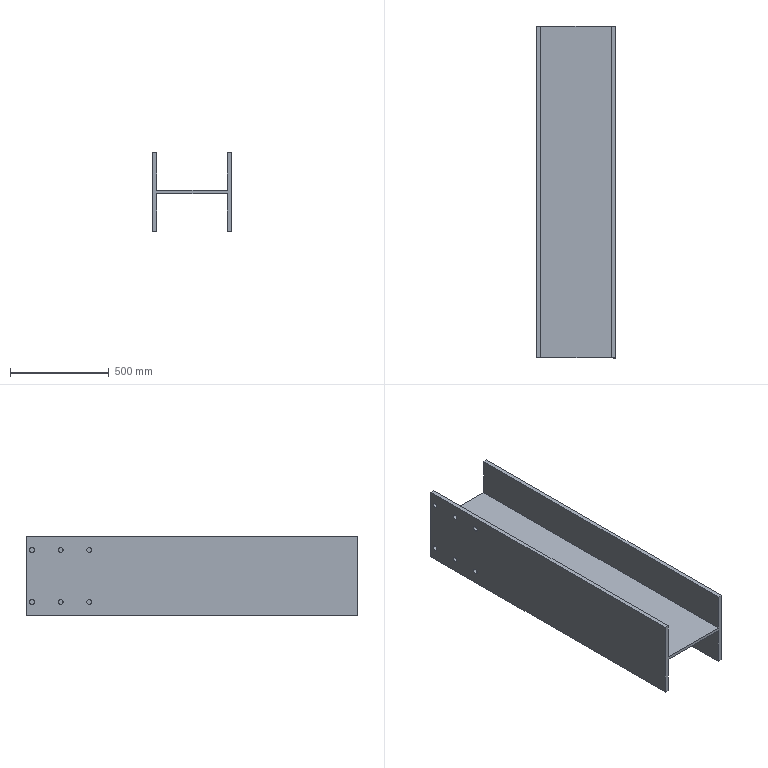Component | SolidWorks | I-Beam-5 | 1 solid | 26 faces | box 400 x 1680 x 400 mm | volume 37785190 mm3 | plane 14 | cylinder 12 | commonest cylinder face diameters 25 x12 | material Plain Carbon Steel
build123d program:
from build123d import *

# Parameters (mm, degrees)
BOSS_EXTRUDE1_DEPTH = 1680
CUT_EXTRUDE1_REACH  = 1774.682
SKETCH2_R           = 12.5


with BuildPart() as part:
    # Sketch1 → Boss-Extrude1 (new body)
    with BuildSketch(Plane(origin=(0, 0, 0), x_dir=(1, 0, 0), z_dir=(0, 1, 0))):
        Polygon((0, 0), (0, 400), (21, 400), (21, 208), (379, 208), (379, 400), (400, 400), (400, 0), (379, 0), (379, 192), (21, 192), (21, 0), align=None)
    extrude(amount=BOSS_EXTRUDE1_DEPTH)

    # Sketch2 → Cut-Extrude1 (cut, up to next)
    with BuildSketch(Plane(origin=(400, 0, 0), x_dir=(0, 0, -1), z_dir=(1, 0, 0)), mode=Mode.PRIVATE) as cut_extrude1_sk1:
        with Locations((68.182, 1650)):
            Circle(SKETCH2_R)
    cut_extrude1_tool1 = extrude(cut_extrude1_sk1.sketch, amount=-CUT_EXTRUDE1_REACH, mode=Mode.PRIVATE) & part.part
    # Sketch2 → Cut-Extrude1 (cut, up to next)
    with BuildSketch(Plane(origin=(400, 0, 0), x_dir=(0, 0, -1), z_dir=(1, 0, 0)), mode=Mode.PRIVATE) as cut_extrude1_sk2:
        with Locations((68.182, 1505)):
            Circle(SKETCH2_R)
    cut_extrude1_tool2 = extrude(cut_extrude1_sk2.sketch, amount=-CUT_EXTRUDE1_REACH, mode=Mode.PRIVATE) & part.part
    # Sketch2 → Cut-Extrude1 (cut, up to next)
    with BuildSketch(Plane(origin=(400, 0, 0), x_dir=(0, 0, -1), z_dir=(1, 0, 0)), mode=Mode.PRIVATE) as cut_extrude1_sk3:
        with Locations((331.818, 1360)):
            Circle(SKETCH2_R)
    cut_extrude1_tool3 = extrude(cut_extrude1_sk3.sketch, amount=-CUT_EXTRUDE1_REACH, mode=Mode.PRIVATE) & part.part
    # Sketch2 → Cut-Extrude1 (cut, up to next)
    with BuildSketch(Plane(origin=(400, 0, 0), x_dir=(0, 0, -1), z_dir=(1, 0, 0)), mode=Mode.PRIVATE) as cut_extrude1_sk4:
        with Locations((331.818, 1505)):
            Circle(SKETCH2_R)
    cut_extrude1_tool4 = extrude(cut_extrude1_sk4.sketch, amount=-CUT_EXTRUDE1_REACH, mode=Mode.PRIVATE) & part.part
    # Sketch2 → Cut-Extrude1 (cut, up to next)
    with BuildSketch(Plane(origin=(400, 0, 0), x_dir=(0, 0, -1), z_dir=(1, 0, 0)), mode=Mode.PRIVATE) as cut_extrude1_sk5:
        with Locations((331.818, 1650)):
            Circle(SKETCH2_R)
    cut_extrude1_tool5 = extrude(cut_extrude1_sk5.sketch, amount=-CUT_EXTRUDE1_REACH, mode=Mode.PRIVATE) & part.part
    # Sketch2 → Cut-Extrude1 (cut, up to next)
    with BuildSketch(Plane(origin=(400, 0, 0), x_dir=(0, 0, -1), z_dir=(1, 0, 0)), mode=Mode.PRIVATE) as cut_extrude1_sk6:
        with Locations((68.182, 1360)):
            Circle(SKETCH2_R)
    cut_extrude1_tool6 = extrude(cut_extrude1_sk6.sketch, amount=-CUT_EXTRUDE1_REACH, mode=Mode.PRIVATE) & part.part
    add(cut_extrude1_tool1.solids().sort_by_distance((400, 1650, -68.182))[0], mode=Mode.SUBTRACT)
    add(cut_extrude1_tool2.solids().sort_by_distance((400, 1505, -68.182))[0], mode=Mode.SUBTRACT)
    add(cut_extrude1_tool3.solids().sort_by_distance((400, 1360, -331.818))[0], mode=Mode.SUBTRACT)
    add(cut_extrude1_tool4.solids().sort_by_distance((400, 1505, -331.818))[0], mode=Mode.SUBTRACT)
    add(cut_extrude1_tool5.solids().sort_by_distance((400, 1650, -331.818))[0], mode=Mode.SUBTRACT)
    add(cut_extrude1_tool6.solids().sort_by_distance((400, 1360, -68.182))[0], mode=Mode.SUBTRACT)


solid = part.part

# Placed as in the assembly
solid = solid.moved(Location((17054.937, 1194.803, 1655.287), (-180, 0, 180)))
STEP:
#1=COLOUR_RGB('',0.7922,0.8196,0.9333);
#2=FILL_AREA_STYLE_COLOUR('',#1);
#3=FILL_AREA_STYLE('',(#2));
#4=SURFACE_STYLE_FILL_AREA(#3);
#5=SURFACE_SIDE_STYLE('',(#4));
#6=SURFACE_STYLE_USAGE(.BOTH.,#5);
#7=PRESENTATION_STYLE_ASSIGNMENT((#6));
#8=CARTESIAN_POINT('',(656.533,100.583,68.345));
#9=VERTEX_POINT('',#8);
#10=CARTESIAN_POINT('',(656.533,100.583,67.361));
#11=VERTEX_POINT('',#10);
#12=CARTESIAN_POINT('',(656.533,100.583,67.853));
#13=DIRECTION('',(1.,-0.,-0.));
#14=DIRECTION('',(0.,0.,1.));
#15=AXIS2_PLACEMENT_3D('',#12,#13,#14);
#16=CIRCLE('',#15,0.4921);
#17=EDGE_CURVE('',#9,#11,#16,.T.);
#18=ORIENTED_EDGE('',*,*,#17,.T.);
#19=CARTESIAN_POINT('',(655.706,100.583,67.361));
#20=VERTEX_POINT('',#19);
#21=CARTESIAN_POINT('',(671.454,100.583,67.361));
#22=DIRECTION('',(-1.,0.,0.));
#23=VECTOR('',#22,39.37);
#24=LINE('',#21,#23);
#25=EDGE_CURVE('',#11,#20,#24,.T.);
#26=ORIENTED_EDGE('',*,*,#25,.T.);
#27=CARTESIAN_POINT('',(655.706,100.583,68.345));
#28=VERTEX_POINT('',#27);
#29=CARTESIAN_POINT('',(655.706,100.583,67.853));
#30=DIRECTION('',(-1.,0.,0.));
#31=DIRECTION('',(0.,0.,1.));
#32=AXIS2_PLACEMENT_3D('',#29,#30,#31);
#33=CIRCLE('',#32,0.4921);
#34=EDGE_CURVE('',#20,#28,#33,.T.);
#35=ORIENTED_EDGE('',*,*,#34,.T.);
#36=CARTESIAN_POINT('',(671.454,100.583,68.345));
#37=DIRECTION('',(-1.,0.,0.));
#38=VECTOR('',#37,39.37);
#39=LINE('',#36,#38);
#40=EDGE_CURVE('',#9,#28,#39,.T.);
#41=ORIENTED_EDGE('',*,*,#40,.F.);
#42=EDGE_LOOP('',(#18,#26,#35,#41));
#43=FACE_OUTER_BOUND('',#42,.T.);
#44=CARTESIAN_POINT('',(671.454,100.583,67.853));
#45=DIRECTION('',(-1.,0.,0.));
#46=DIRECTION('',(0.,0.,1.));
#47=AXIS2_PLACEMENT_3D('',#44,#45,#46);
#48=CYLINDRICAL_SURFACE('',#47,0.4921);
#49=ADVANCED_FACE('',(#43),#48,.F.);
#50=CARTESIAN_POINT('',(656.533,106.291,68.345));
#51=VERTEX_POINT('',#50);
#52=CARTESIAN_POINT('',(656.533,106.291,67.361));
#53=VERTEX_POINT('',#52);
#54=CARTESIAN_POINT('',(656.533,106.291,67.853));
#55=DIRECTION('',(1.,-0.,-0.));
#56=DIRECTION('',(0.,0.,1.));
#57=AXIS2_PLACEMENT_3D('',#54,#55,#56);
#58=CIRCLE('',#57,0.4921);
#59=EDGE_CURVE('',#51,#53,#58,.T.);
#60=ORIENTED_EDGE('',*,*,#59,.T.);
#61=CARTESIAN_POINT('',(655.706,106.291,67.361));
#62=VERTEX_POINT('',#61);
#63=CARTESIAN_POINT('',(671.454,106.291,67.361));
#64=DIRECTION('',(-1.,0.,0.));
#65=VECTOR('',#64,39.37);
#66=LINE('',#63,#65);
#67=EDGE_CURVE('',#53,#62,#66,.T.);
#68=ORIENTED_EDGE('',*,*,#67,.T.);
#69=CARTESIAN_POINT('',(655.706,106.291,68.345));
#70=VERTEX_POINT('',#69);
#71=CARTESIAN_POINT('',(655.706,106.291,67.853));
#72=DIRECTION('',(-1.,0.,0.));
#73=DIRECTION('',(0.,0.,1.));
#74=AXIS2_PLACEMENT_3D('',#71,#72,#73);
#75=CIRCLE('',#74,0.4921);
#76=EDGE_CURVE('',#62,#70,#75,.T.);
#77=ORIENTED_EDGE('',*,*,#76,.T.);
#78=CARTESIAN_POINT('',(671.454,106.291,68.345));
#79=DIRECTION('',(-1.,0.,0.));
#80=VECTOR('',#79,39.37);
#81=LINE('',#78,#80);
#82=EDGE_CURVE('',#51,#70,#81,.T.);
#83=ORIENTED_EDGE('',*,*,#82,.F.);
#84=EDGE_LOOP('',(#60,#68,#77,#83));
#85=FACE_OUTER_BOUND('',#84,.T.);
#86=CARTESIAN_POINT('',(671.454,106.291,67.853));
#87=DIRECTION('',(-1.,0.,0.));
#88=DIRECTION('',(0.,0.,1.));
#89=AXIS2_PLACEMENT_3D('',#86,#87,#88);
#90=CYLINDRICAL_SURFACE('',#89,0.4921);
#91=ADVANCED_FACE('',(#85),#90,.F.);
#92=CARTESIAN_POINT('',(656.533,112.,68.345));
#93=VERTEX_POINT('',#92);
#94=CARTESIAN_POINT('',(656.533,112.,67.361));
#95=VERTEX_POINT('',#94);
#96=CARTESIAN_POINT('',(656.533,112.,67.853));
#97=DIRECTION('',(1.,-0.,-0.));
#98=DIRECTION('',(0.,0.,1.));
#99=AXIS2_PLACEMENT_3D('',#96,#97,#98);
#100=CIRCLE('',#99,0.4921);
#101=EDGE_CURVE('',#93,#95,#100,.T.);
#102=ORIENTED_EDGE('',*,*,#101,.T.);
#103=CARTESIAN_POINT('',(655.706,112.,67.361));
#104=VERTEX_POINT('',#103);
#105=CARTESIAN_POINT('',(671.454,112.,67.361));
#106=DIRECTION('',(-1.,0.,0.));
#107=VECTOR('',#106,39.37);
#108=LINE('',#105,#107);
#109=EDGE_CURVE('',#95,#104,#108,.T.);
#110=ORIENTED_EDGE('',*,*,#109,.T.);
#111=CARTESIAN_POINT('',(655.706,112.,68.345));
#112=VERTEX_POINT('',#111);
#113=CARTESIAN_POINT('',(655.706,112.,67.853));
#114=DIRECTION('',(-1.,0.,0.));
#115=DIRECTION('',(0.,0.,1.));
#116=AXIS2_PLACEMENT_3D('',#113,#114,#115);
#117=CIRCLE('',#116,0.4921);
#118=EDGE_CURVE('',#104,#112,#117,.T.);
#119=ORIENTED_EDGE('',*,*,#118,.T.);
#120=CARTESIAN_POINT('',(671.454,112.,68.345));
#121=DIRECTION('',(-1.,0.,0.));
#122=VECTOR('',#121,39.37);
#123=LINE('',#120,#122);
#124=EDGE_CURVE('',#93,#112,#123,.T.);
#125=ORIENTED_EDGE('',*,*,#124,.F.);
#126=EDGE_LOOP('',(#102,#110,#119,#125));
#127=FACE_OUTER_BOUND('',#126,.T.);
#128=CARTESIAN_POINT('',(671.454,112.,67.853));
#129=DIRECTION('',(-1.,0.,0.));
#130=DIRECTION('',(0.,0.,1.));
#131=AXIS2_PLACEMENT_3D('',#128,#129,#130);
#132=CYLINDRICAL_SURFACE('',#131,0.4921);
#133=ADVANCED_FACE('',(#127),#132,.F.);
#134=CARTESIAN_POINT('',(656.533,112.,78.725));
#135=VERTEX_POINT('',#134);
#136=CARTESIAN_POINT('',(656.533,112.,77.74));
#137=VERTEX_POINT('',#136);
#138=CARTESIAN_POINT('',(656.533,112.,78.232));
#139=DIRECTION('',(1.,-0.,-0.));
#140=DIRECTION('',(0.,0.,1.));
#141=AXIS2_PLACEMENT_3D('',#138,#139,#140);
#142=CIRCLE('',#141,0.4921);
#143=EDGE_CURVE('',#135,#137,#142,.T.);
#144=ORIENTED_EDGE('',*,*,#143,.T.);
#145=CARTESIAN_POINT('',(655.706,112.,77.74));
#146=VERTEX_POINT('',#145);
#147=CARTESIAN_POINT('',(671.454,112.,77.74));
#148=DIRECTION('',(-1.,0.,0.));
#149=VECTOR('',#148,39.37);
#150=LINE('',#147,#149);
#151=EDGE_CURVE('',#137,#146,#150,.T.);
#152=ORIENTED_EDGE('',*,*,#151,.T.);
#153=CARTESIAN_POINT('',(655.706,112.,78.725));
#154=VERTEX_POINT('',#153);
#155=CARTESIAN_POINT('',(655.706,112.,78.232));
#156=DIRECTION('',(-1.,0.,0.));
#157=DIRECTION('',(0.,0.,1.));
#158=AXIS2_PLACEMENT_3D('',#155,#156,#157);
#159=CIRCLE('',#158,0.4921);
#160=EDGE_CURVE('',#146,#154,#159,.T.);
#161=ORIENTED_EDGE('',*,*,#160,.T.);
#162=CARTESIAN_POINT('',(671.454,112.,78.725));
#163=DIRECTION('',(-1.,0.,0.));
#164=VECTOR('',#163,39.37);
#165=LINE('',#162,#164);
#166=EDGE_CURVE('',#135,#154,#165,.T.);
#167=ORIENTED_EDGE('',*,*,#166,.F.);
#168=EDGE_LOOP('',(#144,#152,#161,#167));
#169=FACE_OUTER_BOUND('',#168,.T.);
#170=CARTESIAN_POINT('',(671.454,112.,78.232));
#171=DIRECTION('',(-1.,0.,0.));
#172=DIRECTION('',(0.,0.,1.));
#173=AXIS2_PLACEMENT_3D('',#170,#171,#172);
#174=CYLINDRICAL_SURFACE('',#173,0.4921);
#175=ADVANCED_FACE('',(#169),#174,.F.);
#176=CARTESIAN_POINT('',(656.533,106.291,78.725));
#177=VERTEX_POINT('',#176);
#178=CARTESIAN_POINT('',(656.533,106.291,77.74));
#179=VERTEX_POINT('',#178);
#180=CARTESIAN_POINT('',(656.533,106.291,78.232));
#181=DIRECTION('',(1.,-0.,-0.));
#182=DIRECTION('',(0.,0.,1.));
#183=AXIS2_PLACEMENT_3D('',#180,#181,#182);
#184=CIRCLE('',#183,0.4921);
#185=EDGE_CURVE('',#177,#179,#184,.T.);
#186=ORIENTED_EDGE('',*,*,#185,.T.);
#187=CARTESIAN_POINT('',(655.706,106.291,77.74));
#188=VERTEX_POINT('',#187);
#189=CARTESIAN_POINT('',(671.454,106.291,77.74));
#190=DIRECTION('',(-1.,0.,0.));
#191=VECTOR('',#190,39.37);
#192=LINE('',#189,#191);
#193=EDGE_CURVE('',#179,#188,#192,.T.);
#194=ORIENTED_EDGE('',*,*,#193,.T.);
#195=CARTESIAN_POINT('',(655.706,106.291,78.725));
#196=VERTEX_POINT('',#195);
#197=CARTESIAN_POINT('',(655.706,106.291,78.232));
#198=DIRECTION('',(-1.,0.,0.));
#199=DIRECTION('',(0.,0.,1.));
#200=AXIS2_PLACEMENT_3D('',#197,#198,#199);
#201=CIRCLE('',#200,0.4921);
#202=EDGE_CURVE('',#188,#196,#201,.T.);
#203=ORIENTED_EDGE('',*,*,#202,.T.);
#204=CARTESIAN_POINT('',(671.454,106.291,78.725));
#205=DIRECTION('',(-1.,0.,0.));
#206=VECTOR('',#205,39.37);
#207=LINE('',#204,#206);
#208=EDGE_CURVE('',#177,#196,#207,.T.);
#209=ORIENTED_EDGE('',*,*,#208,.F.);
#210=EDGE_LOOP('',(#186,#194,#203,#209));
#211=FACE_OUTER_BOUND('',#210,.T.);
#212=CARTESIAN_POINT('',(671.454,106.291,78.232));
#213=DIRECTION('',(-1.,0.,0.));
#214=DIRECTION('',(0.,0.,1.));
#215=AXIS2_PLACEMENT_3D('',#212,#213,#214);
#216=CYLINDRICAL_SURFACE('',#215,0.4921);
#217=ADVANCED_FACE('',(#211),#216,.F.);
#218=CARTESIAN_POINT('',(656.533,100.583,78.725));
#219=VERTEX_POINT('',#218);
#220=CARTESIAN_POINT('',(656.533,100.583,77.74));
#221=VERTEX_POINT('',#220);
#222=CARTESIAN_POINT('',(656.533,100.583,78.232));
#223=DIRECTION('',(1.,-0.,-0.));
#224=DIRECTION('',(0.,0.,1.));
#225=AXIS2_PLACEMENT_3D('',#222,#223,#224);
#226=CIRCLE('',#225,0.4921);
#227=EDGE_CURVE('',#219,#221,#226,.T.);
#228=ORIENTED_EDGE('',*,*,#227,.T.);
#229=CARTESIAN_POINT('',(655.706,100.583,77.74));
#230=VERTEX_POINT('',#229);
#231=CARTESIAN_POINT('',(671.454,100.583,77.74));
#232=DIRECTION('',(-1.,0.,0.));
#233=VECTOR('',#232,39.37);
#234=LINE('',#231,#233);
#235=EDGE_CURVE('',#221,#230,#234,.T.);
#236=ORIENTED_EDGE('',*,*,#235,.T.);
#237=CARTESIAN_POINT('',(655.706,100.583,78.725));
#238=VERTEX_POINT('',#237);
#239=CARTESIAN_POINT('',(655.706,100.583,78.232));
#240=DIRECTION('',(-1.,0.,0.));
#241=DIRECTION('',(0.,0.,1.));
#242=AXIS2_PLACEMENT_3D('',#239,#240,#241);
#243=CIRCLE('',#242,0.4921);
#244=EDGE_CURVE('',#230,#238,#243,.T.);
#245=ORIENTED_EDGE('',*,*,#244,.T.);
#246=CARTESIAN_POINT('',(671.454,100.583,78.725));
#247=DIRECTION('',(-1.,0.,0.));
#248=VECTOR('',#247,39.37);
#249=LINE('',#246,#248);
#250=EDGE_CURVE('',#219,#238,#249,.T.);
#251=ORIENTED_EDGE('',*,*,#250,.F.);
#252=EDGE_LOOP('',(#228,#236,#245,#251));
#253=FACE_OUTER_BOUND('',#252,.T.);
#254=CARTESIAN_POINT('',(671.454,100.583,78.232));
#255=DIRECTION('',(-1.,0.,0.));
#256=DIRECTION('',(0.,0.,1.));
#257=AXIS2_PLACEMENT_3D('',#254,#255,#256);
#258=CYLINDRICAL_SURFACE('',#257,0.4921);
#259=ADVANCED_FACE('',(#253),#258,.F.);
#260=CARTESIAN_POINT('',(671.454,47.039,65.169));
#261=VERTEX_POINT('',#260);
#262=CARTESIAN_POINT('',(670.627,47.039,65.169));
#263=VERTEX_POINT('',#262);
#264=CARTESIAN_POINT('',(670.627,47.039,65.169));
#265=DIRECTION('',(-1.,0.,0.));
#266=VECTOR('',#265,39.37);
#267=LINE('',#264,#266);
#268=EDGE_CURVE('',#261,#263,#267,.T.);
#269=ORIENTED_EDGE('',*,*,#268,.T.);
#270=CARTESIAN_POINT('',(670.627,113.181,65.169));
#271=VERTEX_POINT('',#270);
#272=CARTESIAN_POINT('',(670.627,113.181,65.169));
#273=DIRECTION('',(-0.,-1.,0.));
#274=VECTOR('',#273,39.37);
#275=LINE('',#272,#274);
#276=EDGE_CURVE('',#271,#263,#275,.T.);
#277=ORIENTED_EDGE('',*,*,#276,.F.);
#278=CARTESIAN_POINT('',(671.454,113.181,65.169));
#279=VERTEX_POINT('',#278);
#280=CARTESIAN_POINT('',(670.627,113.181,65.169));
#281=DIRECTION('',(-1.,0.,0.));
#282=VECTOR('',#281,39.37);
#283=LINE('',#280,#282);
#284=EDGE_CURVE('',#279,#271,#283,.T.);
#285=ORIENTED_EDGE('',*,*,#284,.F.);
#286=CARTESIAN_POINT('',(671.454,113.181,65.169));
#287=DIRECTION('',(-0.,-1.,0.));
#288=VECTOR('',#287,39.37);
#289=LINE('',#286,#288);
#290=EDGE_CURVE('',#279,#261,#289,.T.);
#291=ORIENTED_EDGE('',*,*,#290,.T.);
#292=EDGE_LOOP('',(#269,#277,#285,#291));
#293=FACE_OUTER_BOUND('',#292,.T.);
#294=CARTESIAN_POINT('',(670.627,113.181,65.169));
#295=DIRECTION('',(0.,-0.,1.));
#296=DIRECTION('',(1.,-0.,-0.));
#297=AXIS2_PLACEMENT_3D('',#294,#295,#296);
#298=PLANE('',#297);
#299=ADVANCED_FACE('',(#293),#298,.F.);
#300=CARTESIAN_POINT('',(670.627,47.039,72.728));
#301=VERTEX_POINT('',#300);
#302=CARTESIAN_POINT('',(670.627,47.039,72.728));
#303=DIRECTION('',(0.,-0.,1.));
#304=VECTOR('',#303,39.37);
#305=LINE('',#302,#304);
#306=EDGE_CURVE('',#263,#301,#305,.T.);
#307=ORIENTED_EDGE('',*,*,#306,.T.);
#308=CARTESIAN_POINT('',(670.627,113.181,72.728));
#309=VERTEX_POINT('',#308);
#310=CARTESIAN_POINT('',(670.627,113.181,72.728));
#311=DIRECTION('',(-0.,-1.,0.));
#312=VECTOR('',#311,39.37);
#313=LINE('',#310,#312);
#314=EDGE_CURVE('',#309,#301,#313,.T.);
#315=ORIENTED_EDGE('',*,*,#314,.F.);
#316=CARTESIAN_POINT('',(670.627,113.181,72.728));
#317=DIRECTION('',(0.,-0.,1.));
#318=VECTOR('',#317,39.37);
#319=LINE('',#316,#318);
#320=EDGE_CURVE('',#271,#309,#319,.T.);
#321=ORIENTED_EDGE('',*,*,#320,.F.);
#322=ORIENTED_EDGE('',*,*,#276,.T.);
#323=EDGE_LOOP('',(#307,#315,#321,#322));
#324=FACE_OUTER_BOUND('',#323,.T.);
#325=CARTESIAN_POINT('',(670.627,113.181,72.728));
#326=DIRECTION('',(1.,-0.,-0.));
#327=DIRECTION('',(-0.,0.,-1.));
#328=AXIS2_PLACEMENT_3D('',#325,#326,#327);
#329=PLANE('',#328);
#330=ADVANCED_FACE('',(#324),#329,.F.);
#331=CARTESIAN_POINT('',(656.533,47.039,72.728));
#332=VERTEX_POINT('',#331);
#333=CARTESIAN_POINT('',(656.533,47.039,72.728));
#334=DIRECTION('',(-1.,0.,0.));
#335=VECTOR('',#334,39.37);
#336=LINE('',#333,#335);
#337=EDGE_CURVE('',#301,#332,#336,.T.);
#338=ORIENTED_EDGE('',*,*,#337,.T.);
#339=CARTESIAN_POINT('',(656.533,113.181,72.728));
#340=VERTEX_POINT('',#339);
#341=CARTESIAN_POINT('',(656.533,113.181,72.728));
#342=DIRECTION('',(-0.,-1.,0.));
#343=VECTOR('',#342,39.37);
#344=LINE('',#341,#343);
#345=EDGE_CURVE('',#340,#332,#344,.T.);
#346=ORIENTED_EDGE('',*,*,#345,.F.);
#347=CARTESIAN_POINT('',(656.533,113.181,72.728));
#348=DIRECTION('',(-1.,0.,0.));
#349=VECTOR('',#348,39.37);
#350=LINE('',#347,#349);
#351=EDGE_CURVE('',#309,#340,#350,.T.);
#352=ORIENTED_EDGE('',*,*,#351,.F.);
#353=ORIENTED_EDGE('',*,*,#314,.T.);
#354=EDGE_LOOP('',(#338,#346,#352,#353));
#355=FACE_OUTER_BOUND('',#354,.T.);
#356=CARTESIAN_POINT('',(656.533,113.181,72.728));
#357=DIRECTION('',(0.,-0.,1.));
#358=DIRECTION('',(1.,-0.,-0.));
#359=AXIS2_PLACEMENT_3D('',#356,#357,#358);
#360=PLANE('',#359);
#361=ADVANCED_FACE('',(#355),#360,.F.);
#362=ORIENTED_EDGE('',*,*,#17,.F.);
#363=CARTESIAN_POINT('',(656.533,100.583,67.853));
#364=DIRECTION('',(1.,-0.,-0.));
#365=DIRECTION('',(0.,0.,1.));
#366=AXIS2_PLACEMENT_3D('',#363,#364,#365);
#367=CIRCLE('',#366,0.4921);
#368=EDGE_CURVE('',#11,#9,#367,.T.);
#369=ORIENTED_EDGE('',*,*,#368,.F.);
#370=EDGE_LOOP('',(#362,#369));
#371=FACE_BOUND('',#370,.T.);
#372=ORIENTED_EDGE('',*,*,#59,.F.);
#373=CARTESIAN_POINT('',(656.533,106.291,67.853));
#374=DIRECTION('',(1.,-0.,-0.));
#375=DIRECTION('',(0.,0.,1.));
#376=AXIS2_PLACEMENT_3D('',#373,#374,#375);
#377=CIRCLE('',#376,0.4921);
#378=EDGE_CURVE('',#53,#51,#377,.T.);
#379=ORIENTED_EDGE('',*,*,#378,.F.);
#380=EDGE_LOOP('',(#372,#379));
#381=FACE_BOUND('',#380,.T.);
#382=ORIENTED_EDGE('',*,*,#101,.F.);
#383=CARTESIAN_POINT('',(656.533,112.,67.853));
#384=DIRECTION('',(1.,-0.,-0.));
#385=DIRECTION('',(0.,0.,1.));
#386=AXIS2_PLACEMENT_3D('',#383,#384,#385);
#387=CIRCLE('',#386,0.4921);
#388=EDGE_CURVE('',#95,#93,#387,.T.);
#389=ORIENTED_EDGE('',*,*,#388,.F.);
#390=EDGE_LOOP('',(#382,#389));
#391=FACE_BOUND('',#390,.T.);
#392=CARTESIAN_POINT('',(656.533,47.039,65.169));
#393=VERTEX_POINT('',#392);
#394=CARTESIAN_POINT('',(656.533,47.039,65.169));
#395=DIRECTION('',(-0.,0.,-1.));
#396=VECTOR('',#395,39.37);
#397=LINE('',#394,#396);
#398=EDGE_CURVE('',#332,#393,#397,.T.);
#399=ORIENTED_EDGE('',*,*,#398,.T.);
#400=CARTESIAN_POINT('',(656.533,113.181,65.169));
#401=VERTEX_POINT('',#400);
#402=CARTESIAN_POINT('',(656.533,113.181,65.169));
#403=DIRECTION('',(-0.,-1.,0.));
#404=VECTOR('',#403,39.37);
#405=LINE('',#402,#404);
#406=EDGE_CURVE('',#401,#393,#405,.T.);
#407=ORIENTED_EDGE('',*,*,#406,.F.);
#408=CARTESIAN_POINT('',(656.533,113.181,65.169));
#409=DIRECTION('',(-0.,0.,-1.));
#410=VECTOR('',#409,39.37);
#411=LINE('',#408,#410);
#412=EDGE_CURVE('',#340,#401,#411,.T.);
#413=ORIENTED_EDGE('',*,*,#412,.F.);
#414=ORIENTED_EDGE('',*,*,#345,.T.);
#415=EDGE_LOOP('',(#399,#407,#413,#414));
#416=FACE_OUTER_BOUND('',#415,.T.);
#417=CARTESIAN_POINT('',(656.533,113.181,65.169));
#418=DIRECTION('',(-1.,0.,0.));
#419=DIRECTION('',(0.,-0.,1.));
#420=AXIS2_PLACEMENT_3D('',#417,#418,#419);
#421=PLANE('',#420);
#422=ADVANCED_FACE('',(#371,#381,#391,#416),#421,.F.);
#423=CARTESIAN_POINT('',(655.706,47.039,65.169));
#424=VERTEX_POINT('',#423);
#425=CARTESIAN_POINT('',(655.706,47.039,65.169));
#426=DIRECTION('',(-1.,0.,0.));
#427=VECTOR('',#426,39.37);
#428=LINE('',#425,#427);
#429=EDGE_CURVE('',#393,#424,#428,.T.);
#430=ORIENTED_EDGE('',*,*,#429,.T.);
#431=CARTESIAN_POINT('',(655.706,113.181,65.169));
#432=VERTEX_POINT('',#431);
#433=CARTESIAN_POINT('',(655.706,113.181,65.169));
#434=DIRECTION('',(-0.,-1.,0.));
#435=VECTOR('',#434,39.37);
#436=LINE('',#433,#435);
#437=EDGE_CURVE('',#432,#424,#436,.T.);
#438=ORIENTED_EDGE('',*,*,#437,.F.);
#439=CARTESIAN_POINT('',(655.706,113.181,65.169));
#440=DIRECTION('',(-1.,0.,0.));
#441=VECTOR('',#440,39.37);
#442=LINE('',#439,#441);
#443=EDGE_CURVE('',#401,#432,#442,.T.);
#444=ORIENTED_EDGE('',*,*,#443,.F.);
#445=ORIENTED_EDGE('',*,*,#406,.T.);
#446=EDGE_LOOP('',(#430,#438,#444,#445));
#447=FACE_OUTER_BOUND('',#446,.T.);
#448=CARTESIAN_POINT('',(655.706,113.181,65.169));
#449=DIRECTION('',(0.,-0.,1.));
#450=DIRECTION('',(1.,-0.,-0.));
#451=AXIS2_PLACEMENT_3D('',#448,#449,#450);
#452=PLANE('',#451);
#453=ADVANCED_FACE('',(#447),#452,.F.);
#454=CARTESIAN_POINT('',(655.706,112.,78.232));
#455=DIRECTION('',(-1.,0.,0.));
#456=DIRECTION('',(0.,0.,1.));
#457=AXIS2_PLACEMENT_3D('',#454,#455,#456);
#458=CIRCLE('',#457,0.4921);
#459=EDGE_CURVE('',#154,#146,#458,.T.);
#460=ORIENTED_EDGE('',*,*,#459,.F.);
#461=ORIENTED_EDGE('',*,*,#160,.F.);
#462=EDGE_LOOP('',(#460,#461));
#463=FACE_BOUND('',#462,.T.);
#464=CARTESIAN_POINT('',(655.706,106.291,78.232));
#465=DIRECTION('',(-1.,0.,0.));
#466=DIRECTION('',(0.,0.,1.));
#467=AXIS2_PLACEMENT_3D('',#464,#465,#466);
#468=CIRCLE('',#467,0.4921);
#469=EDGE_CURVE('',#196,#188,#468,.T.);
#470=ORIENTED_EDGE('',*,*,#469,.F.);
#471=ORIENTED_EDGE('',*,*,#202,.F.);
#472=EDGE_LOOP('',(#470,#471));
#473=FACE_BOUND('',#472,.T.);
#474=CARTESIAN_POINT('',(655.706,100.583,78.232));
#475=DIRECTION('',(-1.,0.,0.));
#476=DIRECTION('',(0.,0.,1.));
#477=AXIS2_PLACEMENT_3D('',#474,#475,#476);
#478=CIRCLE('',#477,0.4921);
#479=EDGE_CURVE('',#238,#230,#478,.T.);
#480=ORIENTED_EDGE('',*,*,#479,.F.);
#481=ORIENTED_EDGE('',*,*,#244,.F.);
#482=EDGE_LOOP('',(#480,#481));
#483=FACE_BOUND('',#482,.T.);
#484=CARTESIAN_POINT('',(655.706,100.583,67.853));
#485=DIRECTION('',(-1.,0.,0.));
#486=DIRECTION('',(0.,0.,1.));
#487=AXIS2_PLACEMENT_3D('',#484,#485,#486);
#488=CIRCLE('',#487,0.4921);
#489=EDGE_CURVE('',#28,#20,#488,.T.);
#490=ORIENTED_EDGE('',*,*,#489,.F.);
#491=ORIENTED_EDGE('',*,*,#34,.F.);
#492=EDGE_LOOP('',(#490,#491));
#493=FACE_BOUND('',#492,.T.);
#494=CARTESIAN_POINT('',(655.706,106.291,67.853));
#495=DIRECTION('',(-1.,0.,0.));
#496=DIRECTION('',(0.,0.,1.));
#497=AXIS2_PLACEMENT_3D('',#494,#495,#496);
#498=CIRCLE('',#497,0.4921);
#499=EDGE_CURVE('',#70,#62,#498,.T.);
#500=ORIENTED_EDGE('',*,*,#499,.F.);
#501=ORIENTED_EDGE('',*,*,#76,.F.);
#502=EDGE_LOOP('',(#500,#501));
#503=FACE_BOUND('',#502,.T.);
#504=CARTESIAN_POINT('',(655.706,112.,67.853));
#505=DIRECTION('',(-1.,0.,0.));
#506=DIRECTION('',(0.,0.,1.));
#507=AXIS2_PLACEMENT_3D('',#504,#505,#506);
#508=CIRCLE('',#507,0.4921);
#509=EDGE_CURVE('',#112,#104,#508,.T.);
#510=ORIENTED_EDGE('',*,*,#509,.F.);
#511=ORIENTED_EDGE('',*,*,#118,.F.);
#512=EDGE_LOOP('',(#510,#511));
#513=FACE_BOUND('',#512,.T.);
#514=CARTESIAN_POINT('',(655.706,47.039,80.917));
#515=VERTEX_POINT('',#514);
#516=CARTESIAN_POINT('',(655.706,47.039,80.917));
#517=DIRECTION('',(0.,-0.,1.));
#518=VECTOR('',#517,39.37);
#519=LINE('',#516,#518);
#520=EDGE_CURVE('',#424,#515,#519,.T.);
#521=ORIENTED_EDGE('',*,*,#520,.T.);
#522=CARTESIAN_POINT('',(655.706,113.181,80.917));
#523=VERTEX_POINT('',#522);
#524=CARTESIAN_POINT('',(655.706,113.181,80.917));
#525=DIRECTION('',(-0.,-1.,0.));
#526=VECTOR('',#525,39.37);
#527=LINE('',#524,#526);
#528=EDGE_CURVE('',#523,#515,#527,.T.);
#529=ORIENTED_EDGE('',*,*,#528,.F.);
#530=CARTESIAN_POINT('',(655.706,113.181,80.917));
#531=DIRECTION('',(0.,-0.,1.));
#532=VECTOR('',#531,39.37);
#533=LINE('',#530,#532);
#534=EDGE_CURVE('',#432,#523,#533,.T.);
#535=ORIENTED_EDGE('',*,*,#534,.F.);
#536=ORIENTED_EDGE('',*,*,#437,.T.);
#537=EDGE_LOOP('',(#521,#529,#535,#536));
#538=FACE_OUTER_BOUND('',#537,.T.);
#539=CARTESIAN_POINT('',(655.706,113.181,80.917));
#540=DIRECTION('',(1.,-0.,-0.));
#541=DIRECTION('',(-0.,0.,-1.));
#542=AXIS2_PLACEMENT_3D('',#539,#540,#541);
#543=PLANE('',#542);
#544=ADVANCED_FACE('',(#463,#473,#483,#493,#503,#513,#538),#543,.F.);
#545=CARTESIAN_POINT('',(656.533,47.039,80.917));
#546=VERTEX_POINT('',#545);
#547=CARTESIAN_POINT('',(656.533,47.039,80.917));
#548=DIRECTION('',(1.,-0.,-0.));
#549=VECTOR('',#548,39.37);
#550=LINE('',#547,#549);
#551=EDGE_CURVE('',#515,#546,#550,.T.);
#552=ORIENTED_EDGE('',*,*,#551,.T.);
#553=CARTESIAN_POINT('',(656.533,113.181,80.917));
#554=VERTEX_POINT('',#553);
#555=CARTESIAN_POINT('',(656.533,113.181,80.917));
#556=DIRECTION('',(-0.,-1.,0.));
#557=VECTOR('',#556,39.37);
#558=LINE('',#555,#557);
#559=EDGE_CURVE('',#554,#546,#558,.T.);
#560=ORIENTED_EDGE('',*,*,#559,.F.);
#561=CARTESIAN_POINT('',(656.533,113.181,80.917));
#562=DIRECTION('',(1.,-0.,-0.));
#563=VECTOR('',#562,39.37);
#564=LINE('',#561,#563);
#565=EDGE_CURVE('',#523,#554,#564,.T.);
#566=ORIENTED_EDGE('',*,*,#565,.F.);
#567=ORIENTED_EDGE('',*,*,#528,.T.);
#568=EDGE_LOOP('',(#552,#560,#566,#567));
#569=FACE_OUTER_BOUND('',#568,.T.);
#570=CARTESIAN_POINT('',(656.533,113.181,80.917));
#571=DIRECTION('',(-0.,0.,-1.));
#572=DIRECTION('',(-1.,0.,0.));
#573=AXIS2_PLACEMENT_3D('',#570,#571,#572);
#574=PLANE('',#573);
#575=ADVANCED_FACE('',(#569),#574,.F.);
#576=ORIENTED_EDGE('',*,*,#143,.F.);
#577=CARTESIAN_POINT('',(656.533,112.,78.232));
#578=DIRECTION('',(1.,-0.,-0.));
#579=DIRECTION('',(0.,0.,1.));
#580=AXIS2_PLACEMENT_3D('',#577,#578,#579);
#581=CIRCLE('',#580,0.4921);
#582=EDGE_CURVE('',#137,#135,#581,.T.);
#583=ORIENTED_EDGE('',*,*,#582,.F.);
#584=EDGE_LOOP('',(#576,#583));
#585=FACE_BOUND('',#584,.T.);
#586=ORIENTED_EDGE('',*,*,#185,.F.);
#587=CARTESIAN_POINT('',(656.533,106.291,78.232));
#588=DIRECTION('',(1.,-0.,-0.));
#589=DIRECTION('',(0.,0.,1.));
#590=AXIS2_PLACEMENT_3D('',#587,#588,#589);
#591=CIRCLE('',#590,0.4921);
#592=EDGE_CURVE('',#179,#177,#591,.T.);
#593=ORIENTED_EDGE('',*,*,#592,.F.);
#594=EDGE_LOOP('',(#586,#593));
#595=FACE_BOUND('',#594,.T.);
#596=ORIENTED_EDGE('',*,*,#227,.F.);
#597=CARTESIAN_POINT('',(656.533,100.583,78.232));
#598=DIRECTION('',(1.,-0.,-0.));
#599=DIRECTION('',(0.,0.,1.));
#600=AXIS2_PLACEMENT_3D('',#597,#598,#599);
#601=CIRCLE('',#600,0.4921);
#602=EDGE_CURVE('',#221,#219,#601,.T.);
#603=ORIENTED_EDGE('',*,*,#602,.F.);
#604=EDGE_LOOP('',(#596,#603));
#605=FACE_BOUND('',#604,.T.);
#606=CARTESIAN_POINT('',(656.533,47.039,73.358));
#607=VERTEX_POINT('',#606);
#608=CARTESIAN_POINT('',(656.533,47.039,73.358));
#609=DIRECTION('',(-0.,0.,-1.));
#610=VECTOR('',#609,39.37);
#611=LINE('',#608,#610);
#612=EDGE_CURVE('',#546,#607,#611,.T.);
#613=ORIENTED_EDGE('',*,*,#612,.T.);
#614=CARTESIAN_POINT('',(656.533,113.181,73.358));
#615=VERTEX_POINT('',#614);
#616=CARTESIAN_POINT('',(656.533,113.181,73.358));
#617=DIRECTION('',(-0.,-1.,0.));
#618=VECTOR('',#617,39.37);
#619=LINE('',#616,#618);
#620=EDGE_CURVE('',#615,#607,#619,.T.);
#621=ORIENTED_EDGE('',*,*,#620,.F.);
#622=CARTESIAN_POINT('',(656.533,113.181,73.358));
#623=DIRECTION('',(-0.,0.,-1.));
#624=VECTOR('',#623,39.37);
#625=LINE('',#622,#624);
#626=EDGE_CURVE('',#554,#615,#625,.T.);
#627=ORIENTED_EDGE('',*,*,#626,.F.);
#628=ORIENTED_EDGE('',*,*,#559,.T.);
#629=EDGE_LOOP('',(#613,#621,#627,#628));
#630=FACE_OUTER_BOUND('',#629,.T.);
#631=CARTESIAN_POINT('',(656.533,113.181,73.358));
#632=DIRECTION('',(-1.,0.,0.));
#633=DIRECTION('',(0.,-0.,1.));
#634=AXIS2_PLACEMENT_3D('',#631,#632,#633);
#635=PLANE('',#634);
#636=ADVANCED_FACE('',(#585,#595,#605,#630),#635,.F.);
#637=CARTESIAN_POINT('',(670.627,47.039,73.358));
#638=VERTEX_POINT('',#637);
#639=CARTESIAN_POINT('',(670.627,47.039,73.358));
#640=DIRECTION('',(1.,-0.,-0.));
#641=VECTOR('',#640,39.37);
#642=LINE('',#639,#641);
#643=EDGE_CURVE('',#607,#638,#642,.T.);
#644=ORIENTED_EDGE('',*,*,#643,.T.);
#645=CARTESIAN_POINT('',(670.627,113.181,73.358));
#646=VERTEX_POINT('',#645);
#647=CARTESIAN_POINT('',(670.627,113.181,73.358));
#648=DIRECTION('',(-0.,-1.,0.));
#649=VECTOR('',#648,39.37);
#650=LINE('',#647,#649);
#651=EDGE_CURVE('',#646,#638,#650,.T.);
#652=ORIENTED_EDGE('',*,*,#651,.F.);
#653=CARTESIAN_POINT('',(670.627,113.181,73.358));
#654=DIRECTION('',(1.,-0.,-0.));
#655=VECTOR('',#654,39.37);
#656=LINE('',#653,#655);
#657=EDGE_CURVE('',#615,#646,#656,.T.);
#658=ORIENTED_EDGE('',*,*,#657,.F.);
#659=ORIENTED_EDGE('',*,*,#620,.T.);
#660=EDGE_LOOP('',(#644,#652,#658,#659));
#661=FACE_OUTER_BOUND('',#660,.T.);
#662=CARTESIAN_POINT('',(670.627,113.181,73.358));
#663=DIRECTION('',(-0.,0.,-1.));
#664=DIRECTION('',(-1.,0.,0.));
#665=AXIS2_PLACEMENT_3D('',#662,#663,#664);
#666=PLANE('',#665);
#667=ADVANCED_FACE('',(#661),#666,.F.);
#668=CARTESIAN_POINT('',(670.627,47.039,80.917));
#669=VERTEX_POINT('',#668);
#670=CARTESIAN_POINT('',(670.627,47.039,80.917));
#671=DIRECTION('',(0.,-0.,1.));
#672=VECTOR('',#671,39.37);
#673=LINE('',#670,#672);
#674=EDGE_CURVE('',#638,#669,#673,.T.);
#675=ORIENTED_EDGE('',*,*,#674,.T.);
#676=CARTESIAN_POINT('',(670.627,113.181,80.917));
#677=VERTEX_POINT('',#676);
#678=CARTESIAN_POINT('',(670.627,113.181,80.917));
#679=DIRECTION('',(-0.,-1.,0.));
#680=VECTOR('',#679,39.37);
#681=LINE('',#678,#680);
#682=EDGE_CURVE('',#677,#669,#681,.T.);
#683=ORIENTED_EDGE('',*,*,#682,.F.);
#684=CARTESIAN_POINT('',(670.627,113.181,80.917));
#685=DIRECTION('',(0.,-0.,1.));
#686=VECTOR('',#685,39.37);
#687=LINE('',#684,#686);
#688=EDGE_CURVE('',#646,#677,#687,.T.);
#689=ORIENTED_EDGE('',*,*,#688,.F.);
#690=ORIENTED_EDGE('',*,*,#651,.T.);
#691=EDGE_LOOP('',(#675,#683,#689,#690));
#692=FACE_OUTER_BOUND('',#691,.T.);
#693=CARTESIAN_POINT('',(670.627,113.181,80.917));
#694=DIRECTION('',(1.,-0.,-0.));
#695=DIRECTION('',(-0.,0.,-1.));
#696=AXIS2_PLACEMENT_3D('',#693,#694,#695);
#697=PLANE('',#696);
#698=ADVANCED_FACE('',(#692),#697,.F.);
#699=CARTESIAN_POINT('',(671.454,47.039,80.917));
#700=VERTEX_POINT('',#699);
#701=CARTESIAN_POINT('',(671.454,47.039,80.917));
#702=DIRECTION('',(1.,-0.,-0.));
#703=VECTOR('',#702,39.37);
#704=LINE('',#701,#703);
#705=EDGE_CURVE('',#669,#700,#704,.T.);
#706=ORIENTED_EDGE('',*,*,#705,.T.);
#707=CARTESIAN_POINT('',(671.454,113.181,80.917));
#708=VERTEX_POINT('',#707);
#709=CARTESIAN_POINT('',(671.454,113.181,80.917));
#710=DIRECTION('',(-0.,-1.,0.));
#711=VECTOR('',#710,39.37);
#712=LINE('',#709,#711);
#713=EDGE_CURVE('',#708,#700,#712,.T.);
#714=ORIENTED_EDGE('',*,*,#713,.F.);
#715=CARTESIAN_POINT('',(671.454,113.181,80.917));
#716=DIRECTION('',(1.,-0.,-0.));
#717=VECTOR('',#716,39.37);
#718=LINE('',#715,#717);
#719=EDGE_CURVE('',#677,#708,#718,.T.);
#720=ORIENTED_EDGE('',*,*,#719,.F.);
#721=ORIENTED_EDGE('',*,*,#682,.T.);
#722=EDGE_LOOP('',(#706,#714,#720,#721));
#723=FACE_OUTER_BOUND('',#722,.T.);
#724=CARTESIAN_POINT('',(671.454,113.181,80.917));
#725=DIRECTION('',(-0.,0.,-1.));
#726=DIRECTION('',(-1.,0.,0.));
#727=AXIS2_PLACEMENT_3D('',#724,#725,#726);
#728=PLANE('',#727);
#729=ADVANCED_FACE('',(#723),#728,.F.);
#730=CARTESIAN_POINT('',(671.454,47.039,65.169));
#731=DIRECTION('',(-0.,0.,-1.));
#732=VECTOR('',#731,39.37);
#733=LINE('',#730,#732);
#734=EDGE_CURVE('',#700,#261,#733,.T.);
#735=ORIENTED_EDGE('',*,*,#734,.T.);
#736=ORIENTED_EDGE('',*,*,#290,.F.);
#737=CARTESIAN_POINT('',(671.454,113.181,65.169));
#738=DIRECTION('',(-0.,0.,-1.));
#739=VECTOR('',#738,39.37);
#740=LINE('',#737,#739);
#741=EDGE_CURVE('',#708,#279,#740,.T.);
#742=ORIENTED_EDGE('',*,*,#741,.F.);
#743=ORIENTED_EDGE('',*,*,#713,.T.);
#744=EDGE_LOOP('',(#735,#736,#742,#743));
#745=FACE_OUTER_BOUND('',#744,.T.);
#746=CARTESIAN_POINT('',(671.454,113.181,65.169));
#747=DIRECTION('',(-1.,0.,0.));
#748=DIRECTION('',(0.,-0.,1.));
#749=AXIS2_PLACEMENT_3D('',#746,#747,#748);
#750=PLANE('',#749);
#751=ADVANCED_FACE('',(#745),#750,.F.);
#752=ORIENTED_EDGE('',*,*,#284,.T.);
#753=ORIENTED_EDGE('',*,*,#320,.T.);
#754=ORIENTED_EDGE('',*,*,#351,.T.);
#755=ORIENTED_EDGE('',*,*,#412,.T.);
#756=ORIENTED_EDGE('',*,*,#443,.T.);
#757=ORIENTED_EDGE('',*,*,#534,.T.);
#758=ORIENTED_EDGE('',*,*,#565,.T.);
#759=ORIENTED_EDGE('',*,*,#626,.T.);
#760=ORIENTED_EDGE('',*,*,#657,.T.);
#761=ORIENTED_EDGE('',*,*,#688,.T.);
#762=ORIENTED_EDGE('',*,*,#719,.T.);
#763=ORIENTED_EDGE('',*,*,#741,.T.);
#764=EDGE_LOOP('',(#752,#753,#754,#755,#756,#757,#758,#759,#760,#761,#762,#763));
#765=FACE_OUTER_BOUND('',#764,.T.);
#766=CARTESIAN_POINT('',(671.454,113.181,65.169));
#767=DIRECTION('',(-0.,-1.,0.));
#768=DIRECTION('',(0.,-0.,1.));
#769=AXIS2_PLACEMENT_3D('',#766,#767,#768);
#770=PLANE('',#769);
#771=ADVANCED_FACE('',(#765),#770,.F.);
#772=ORIENTED_EDGE('',*,*,#268,.F.);
#773=ORIENTED_EDGE('',*,*,#734,.F.);
#774=ORIENTED_EDGE('',*,*,#705,.F.);
#775=ORIENTED_EDGE('',*,*,#674,.F.);
#776=ORIENTED_EDGE('',*,*,#643,.F.);
#777=ORIENTED_EDGE('',*,*,#612,.F.);
#778=ORIENTED_EDGE('',*,*,#551,.F.);
#779=ORIENTED_EDGE('',*,*,#520,.F.);
#780=ORIENTED_EDGE('',*,*,#429,.F.);
#781=ORIENTED_EDGE('',*,*,#398,.F.);
#782=ORIENTED_EDGE('',*,*,#337,.F.);
#783=ORIENTED_EDGE('',*,*,#306,.F.);
#784=EDGE_LOOP('',(#772,#773,#774,#775,#776,#777,#778,#779,#780,#781,#782,#783));
#785=FACE_OUTER_BOUND('',#784,.T.);
#786=CARTESIAN_POINT('',(671.454,47.039,65.169));
#787=DIRECTION('',(-0.,-1.,0.));
#788=DIRECTION('',(0.,-0.,1.));
#789=AXIS2_PLACEMENT_3D('',#786,#787,#788);
#790=PLANE('',#789);
#791=ADVANCED_FACE('',(#785),#790,.T.);
#792=ORIENTED_EDGE('',*,*,#235,.F.);
#793=ORIENTED_EDGE('',*,*,#602,.T.);
#794=ORIENTED_EDGE('',*,*,#250,.T.);
#795=ORIENTED_EDGE('',*,*,#479,.T.);
#796=EDGE_LOOP('',(#792,#793,#794,#795));
#797=FACE_OUTER_BOUND('',#796,.T.);
#798=CARTESIAN_POINT('',(671.454,100.583,78.232));
#799=DIRECTION('',(-1.,0.,0.));
#800=DIRECTION('',(0.,0.,1.));
#801=AXIS2_PLACEMENT_3D('',#798,#799,#800);
#802=CYLINDRICAL_SURFACE('',#801,0.4921);
#803=ADVANCED_FACE('',(#797),#802,.F.);
#804=ORIENTED_EDGE('',*,*,#193,.F.);
#805=ORIENTED_EDGE('',*,*,#592,.T.);
#806=ORIENTED_EDGE('',*,*,#208,.T.);
#807=ORIENTED_EDGE('',*,*,#469,.T.);
#808=EDGE_LOOP('',(#804,#805,#806,#807));
#809=FACE_OUTER_BOUND('',#808,.T.);
#810=CARTESIAN_POINT('',(671.454,106.291,78.232));
#811=DIRECTION('',(-1.,0.,0.));
#812=DIRECTION('',(0.,0.,1.));
#813=AXIS2_PLACEMENT_3D('',#810,#811,#812);
#814=CYLINDRICAL_SURFACE('',#813,0.4921);
#815=ADVANCED_FACE('',(#809),#814,.F.);
#816=ORIENTED_EDGE('',*,*,#151,.F.);
#817=ORIENTED_EDGE('',*,*,#582,.T.);
#818=ORIENTED_EDGE('',*,*,#166,.T.);
#819=ORIENTED_EDGE('',*,*,#459,.T.);
#820=EDGE_LOOP('',(#816,#817,#818,#819));
#821=FACE_OUTER_BOUND('',#820,.T.);
#822=CARTESIAN_POINT('',(671.454,112.,78.232));
#823=DIRECTION('',(-1.,0.,0.));
#824=DIRECTION('',(0.,0.,1.));
#825=AXIS2_PLACEMENT_3D('',#822,#823,#824);
#826=CYLINDRICAL_SURFACE('',#825,0.4921);
#827=ADVANCED_FACE('',(#821),#826,.F.);
#828=ORIENTED_EDGE('',*,*,#109,.F.);
#829=ORIENTED_EDGE('',*,*,#388,.T.);
#830=ORIENTED_EDGE('',*,*,#124,.T.);
#831=ORIENTED_EDGE('',*,*,#509,.T.);
#832=EDGE_LOOP('',(#828,#829,#830,#831));
#833=FACE_OUTER_BOUND('',#832,.T.);
#834=CARTESIAN_POINT('',(671.454,112.,67.853));
#835=DIRECTION('',(-1.,0.,0.));
#836=DIRECTION('',(0.,0.,1.));
#837=AXIS2_PLACEMENT_3D('',#834,#835,#836);
#838=CYLINDRICAL_SURFACE('',#837,0.4921);
#839=ADVANCED_FACE('',(#833),#838,.F.);
#840=ORIENTED_EDGE('',*,*,#67,.F.);
#841=ORIENTED_EDGE('',*,*,#378,.T.);
#842=ORIENTED_EDGE('',*,*,#82,.T.);
#843=ORIENTED_EDGE('',*,*,#499,.T.);
#844=EDGE_LOOP('',(#840,#841,#842,#843));
#845=FACE_OUTER_BOUND('',#844,.T.);
#846=CARTESIAN_POINT('',(671.454,106.291,67.853));
#847=DIRECTION('',(-1.,0.,0.));
#848=DIRECTION('',(0.,0.,1.));
#849=AXIS2_PLACEMENT_3D('',#846,#847,#848);
#850=CYLINDRICAL_SURFACE('',#849,0.4921);
#851=ADVANCED_FACE('',(#845),#850,.F.);
#852=ORIENTED_EDGE('',*,*,#25,.F.);
#853=ORIENTED_EDGE('',*,*,#368,.T.);
#854=ORIENTED_EDGE('',*,*,#40,.T.);
#855=ORIENTED_EDGE('',*,*,#489,.T.);
#856=EDGE_LOOP('',(#852,#853,#854,#855));
#857=FACE_OUTER_BOUND('',#856,.T.);
#858=CARTESIAN_POINT('',(671.454,100.583,67.853));
#859=DIRECTION('',(-1.,0.,0.));
#860=DIRECTION('',(0.,0.,1.));
#861=AXIS2_PLACEMENT_3D('',#858,#859,#860);
#862=CYLINDRICAL_SURFACE('',#861,0.4921);
#863=ADVANCED_FACE('',(#857),#862,.F.);
#864=CLOSED_SHELL('',(#49,#91,#133,#175,#217,#259,#299,#330,#361,#422,#453,#544,#575,#636,#667,#698,#729,#751,#771,#791,#803,#815,#827,#839,#851,#863));
#865=MANIFOLD_SOLID_BREP('',#864);
#866=STYLED_ITEM('',(#7),#865);
#867=PRESENTATION_LAYER_ASSIGNMENT('','',(#866));
#868=(LENGTH_UNIT()NAMED_UNIT(*)SI_UNIT($,.METRE.));
#869=LENGTH_MEASURE_WITH_UNIT(LENGTH_MEASURE(0.0254),#868);
#870=DIMENSIONAL_EXPONENTS(1.,0.,0.,0.,0.,0.,0.);
#871=(CONVERSION_BASED_UNIT('',#869)LENGTH_UNIT()NAMED_UNIT(#870));
#872=UNCERTAINTY_MEASURE_WITH_UNIT(LENGTH_MEASURE(0.00001),#871,'','');
#873=(NAMED_UNIT(*)PLANE_ANGLE_UNIT()SI_UNIT($,.RADIAN.));
#874=(NAMED_UNIT(*)SI_UNIT($,.STERADIAN.)SOLID_ANGLE_UNIT());
#875=(GEOMETRIC_REPRESENTATION_CONTEXT(3)GLOBAL_UNCERTAINTY_ASSIGNED_CONTEXT((#872))GLOBAL_UNIT_ASSIGNED_CONTEXT((#871,#873,#874))REPRESENTATION_CONTEXT('',''));
#876=MECHANICAL_DESIGN_GEOMETRIC_PRESENTATION_REPRESENTATION('',(#866),#875);
#877=CARTESIAN_POINT('',(0.,0.,0.));
#878=DIRECTION('',(0.,0.,1.));
#879=DIRECTION('',(1.,0.,0.));
#880=AXIS2_PLACEMENT_3D('',#877,#878,#879);
#881=(LENGTH_UNIT()NAMED_UNIT(*)SI_UNIT($,.METRE.));
#882=LENGTH_MEASURE_WITH_UNIT(LENGTH_MEASURE(0.0254),#881);
#883=DIMENSIONAL_EXPONENTS(1.,0.,0.,0.,0.,0.,0.);
#884=(CONVERSION_BASED_UNIT('',#882)LENGTH_UNIT()NAMED_UNIT(#883));
#885=UNCERTAINTY_MEASURE_WITH_UNIT(LENGTH_MEASURE(0.00001),#884,'','');
#886=(NAMED_UNIT(*)PLANE_ANGLE_UNIT()SI_UNIT($,.RADIAN.));
#887=(NAMED_UNIT(*)SI_UNIT($,.STERADIAN.)SOLID_ANGLE_UNIT());
#888=(GEOMETRIC_REPRESENTATION_CONTEXT(3)GLOBAL_UNCERTAINTY_ASSIGNED_CONTEXT((#885))GLOBAL_UNIT_ASSIGNED_CONTEXT((#884,#886,#887))REPRESENTATION_CONTEXT('',''));
#889=ADVANCED_BREP_SHAPE_REPRESENTATION('',(#865,#880),#888);